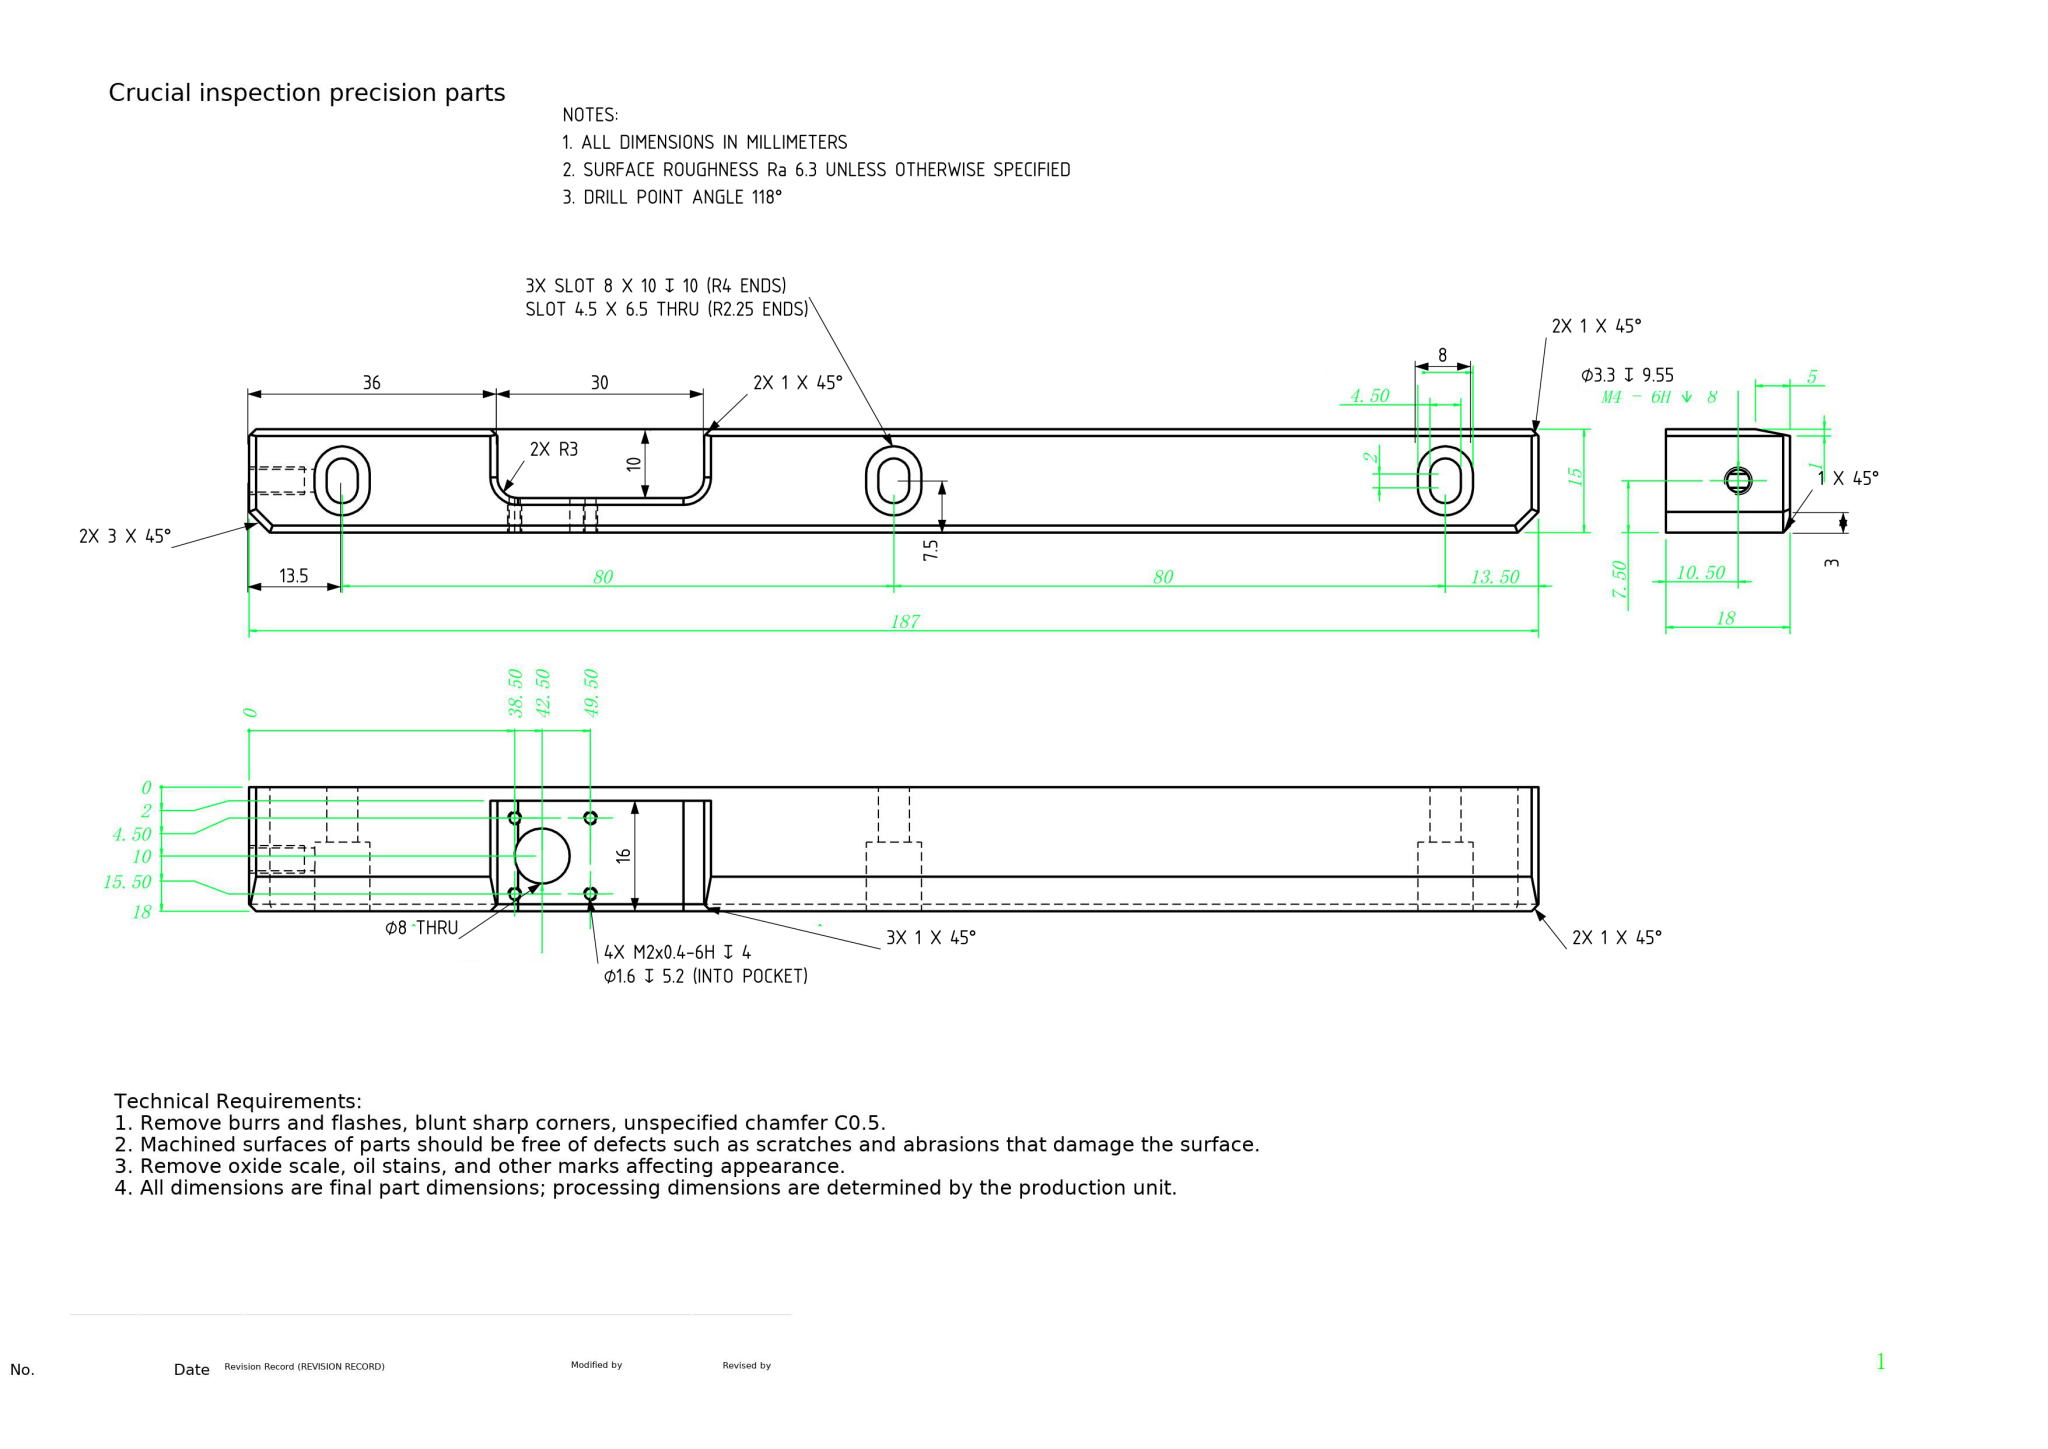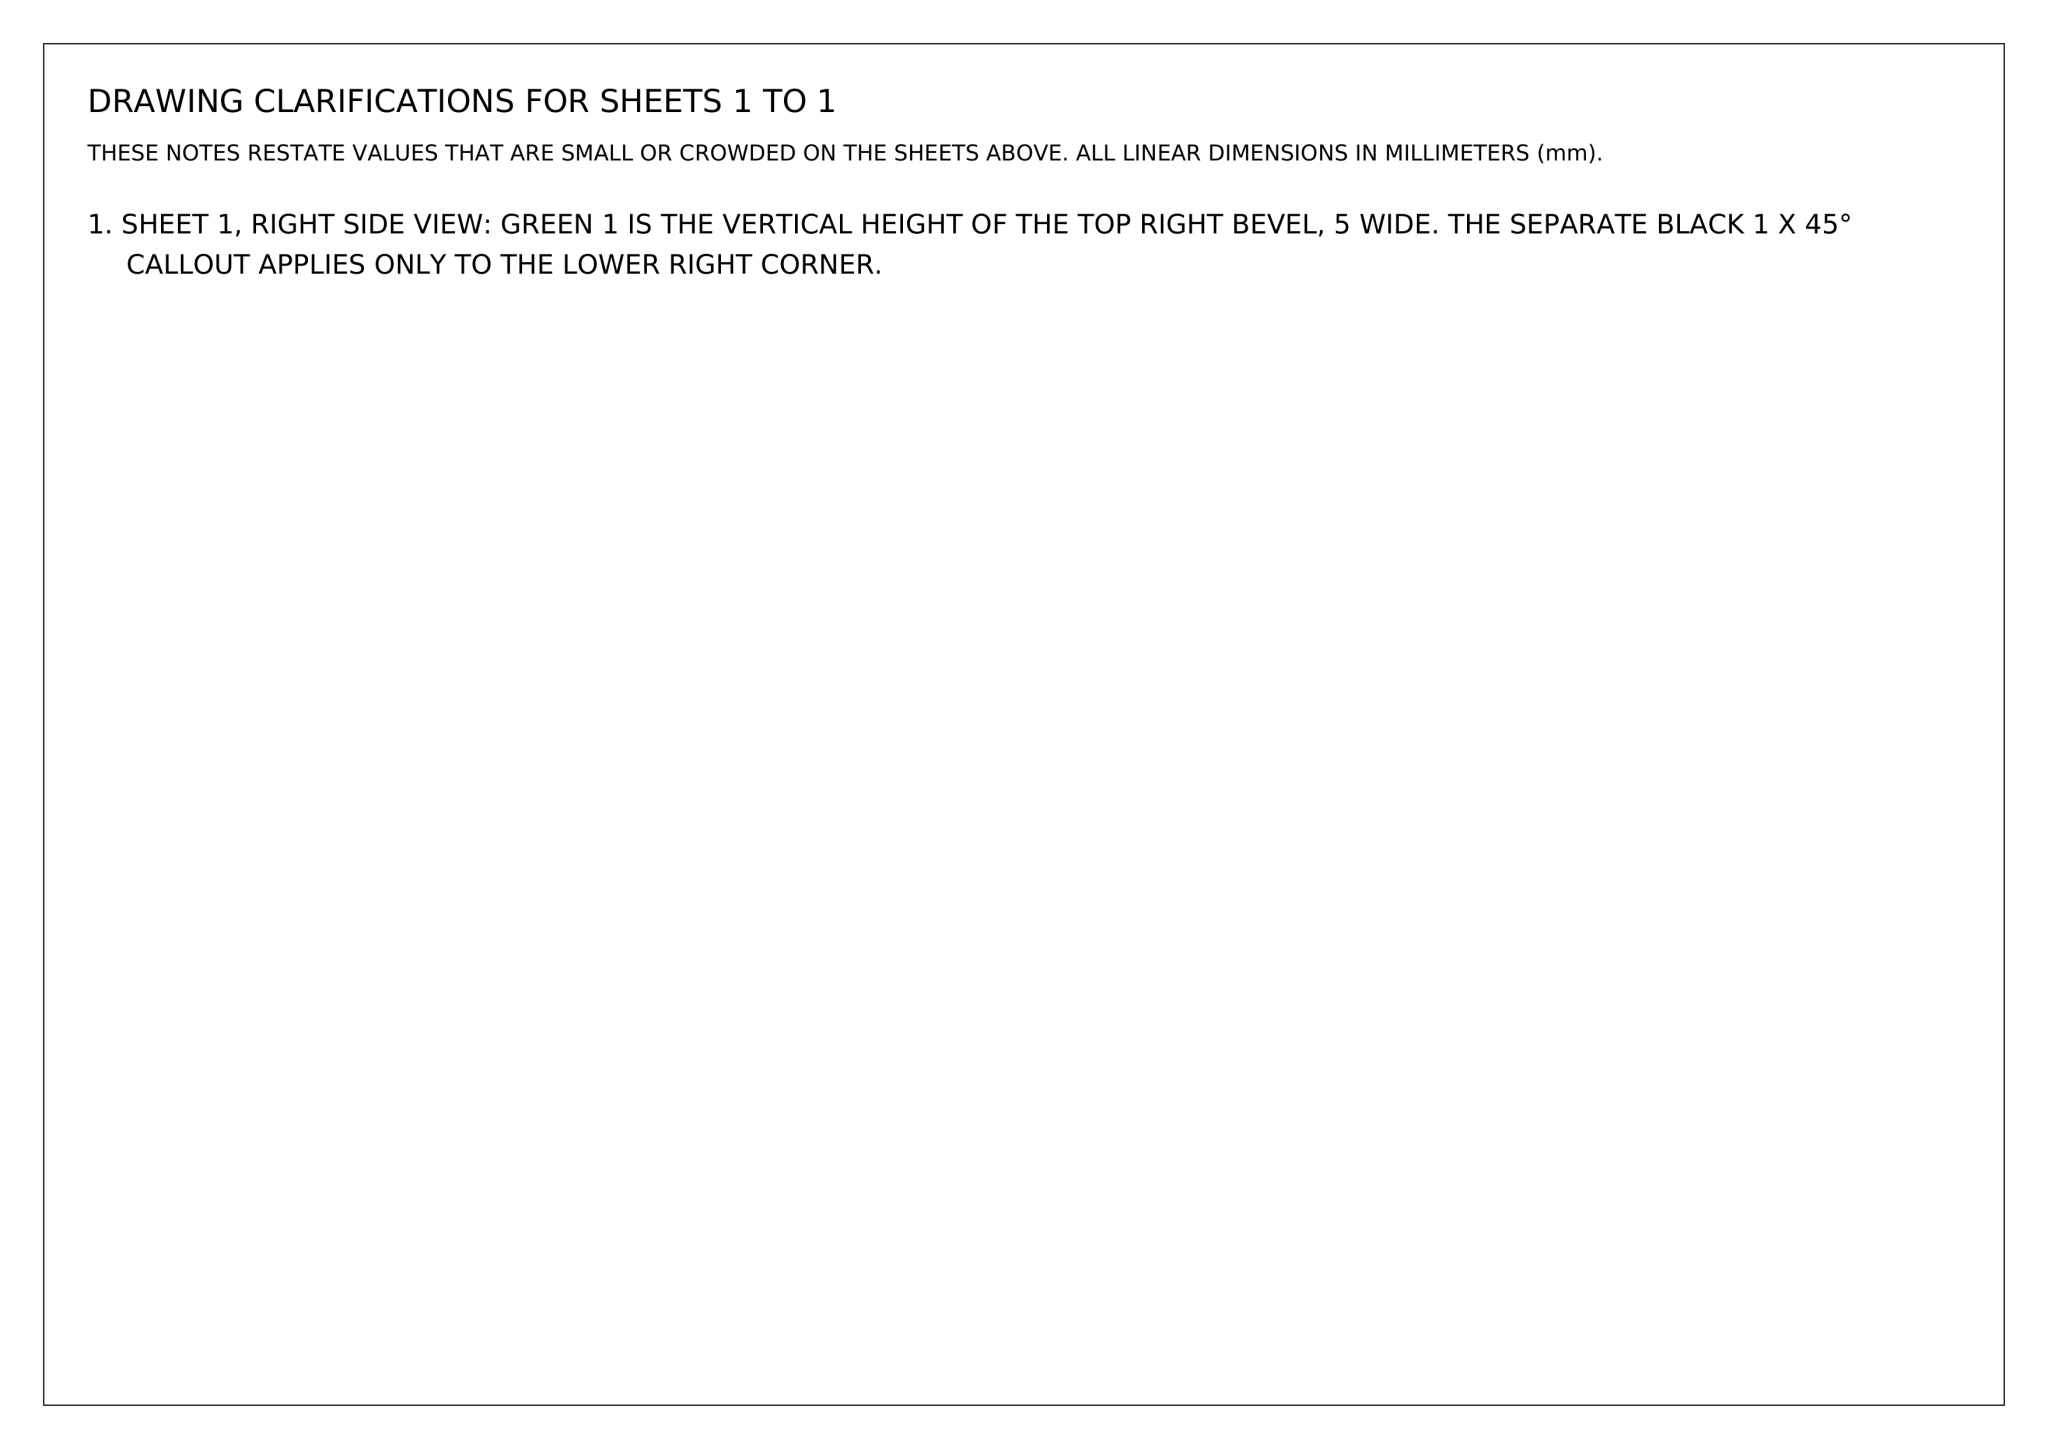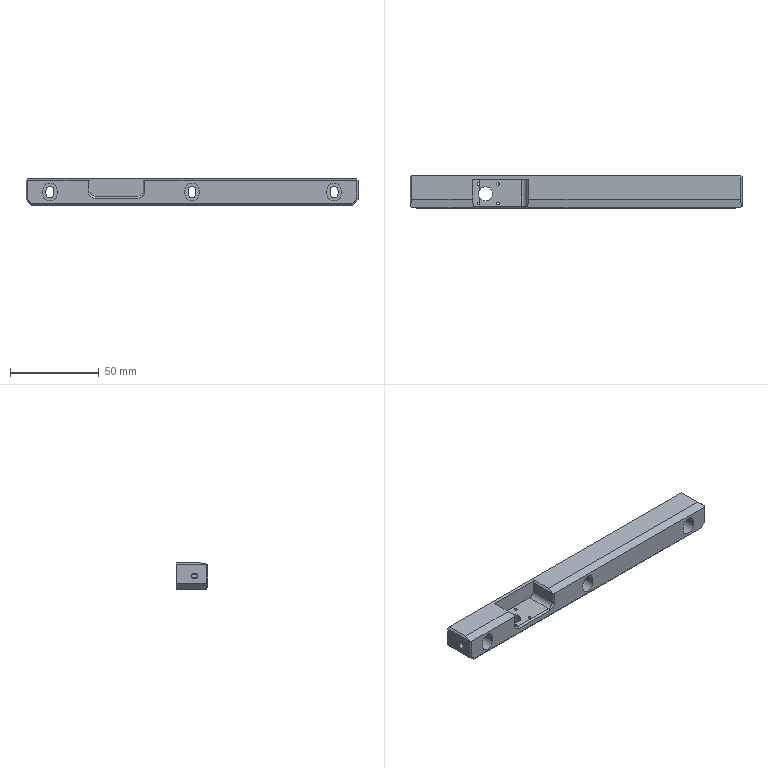Part | NX | mm | 1 solid | 78 faces | box 187 x 18 x 15 mm | volume 42083 mm3 | plane 42 | cylinder 32 | cone 4 | commonest cylinder face diameters 8 x11 4.5 x9 1.6 x8 3.3 x2 6 x2